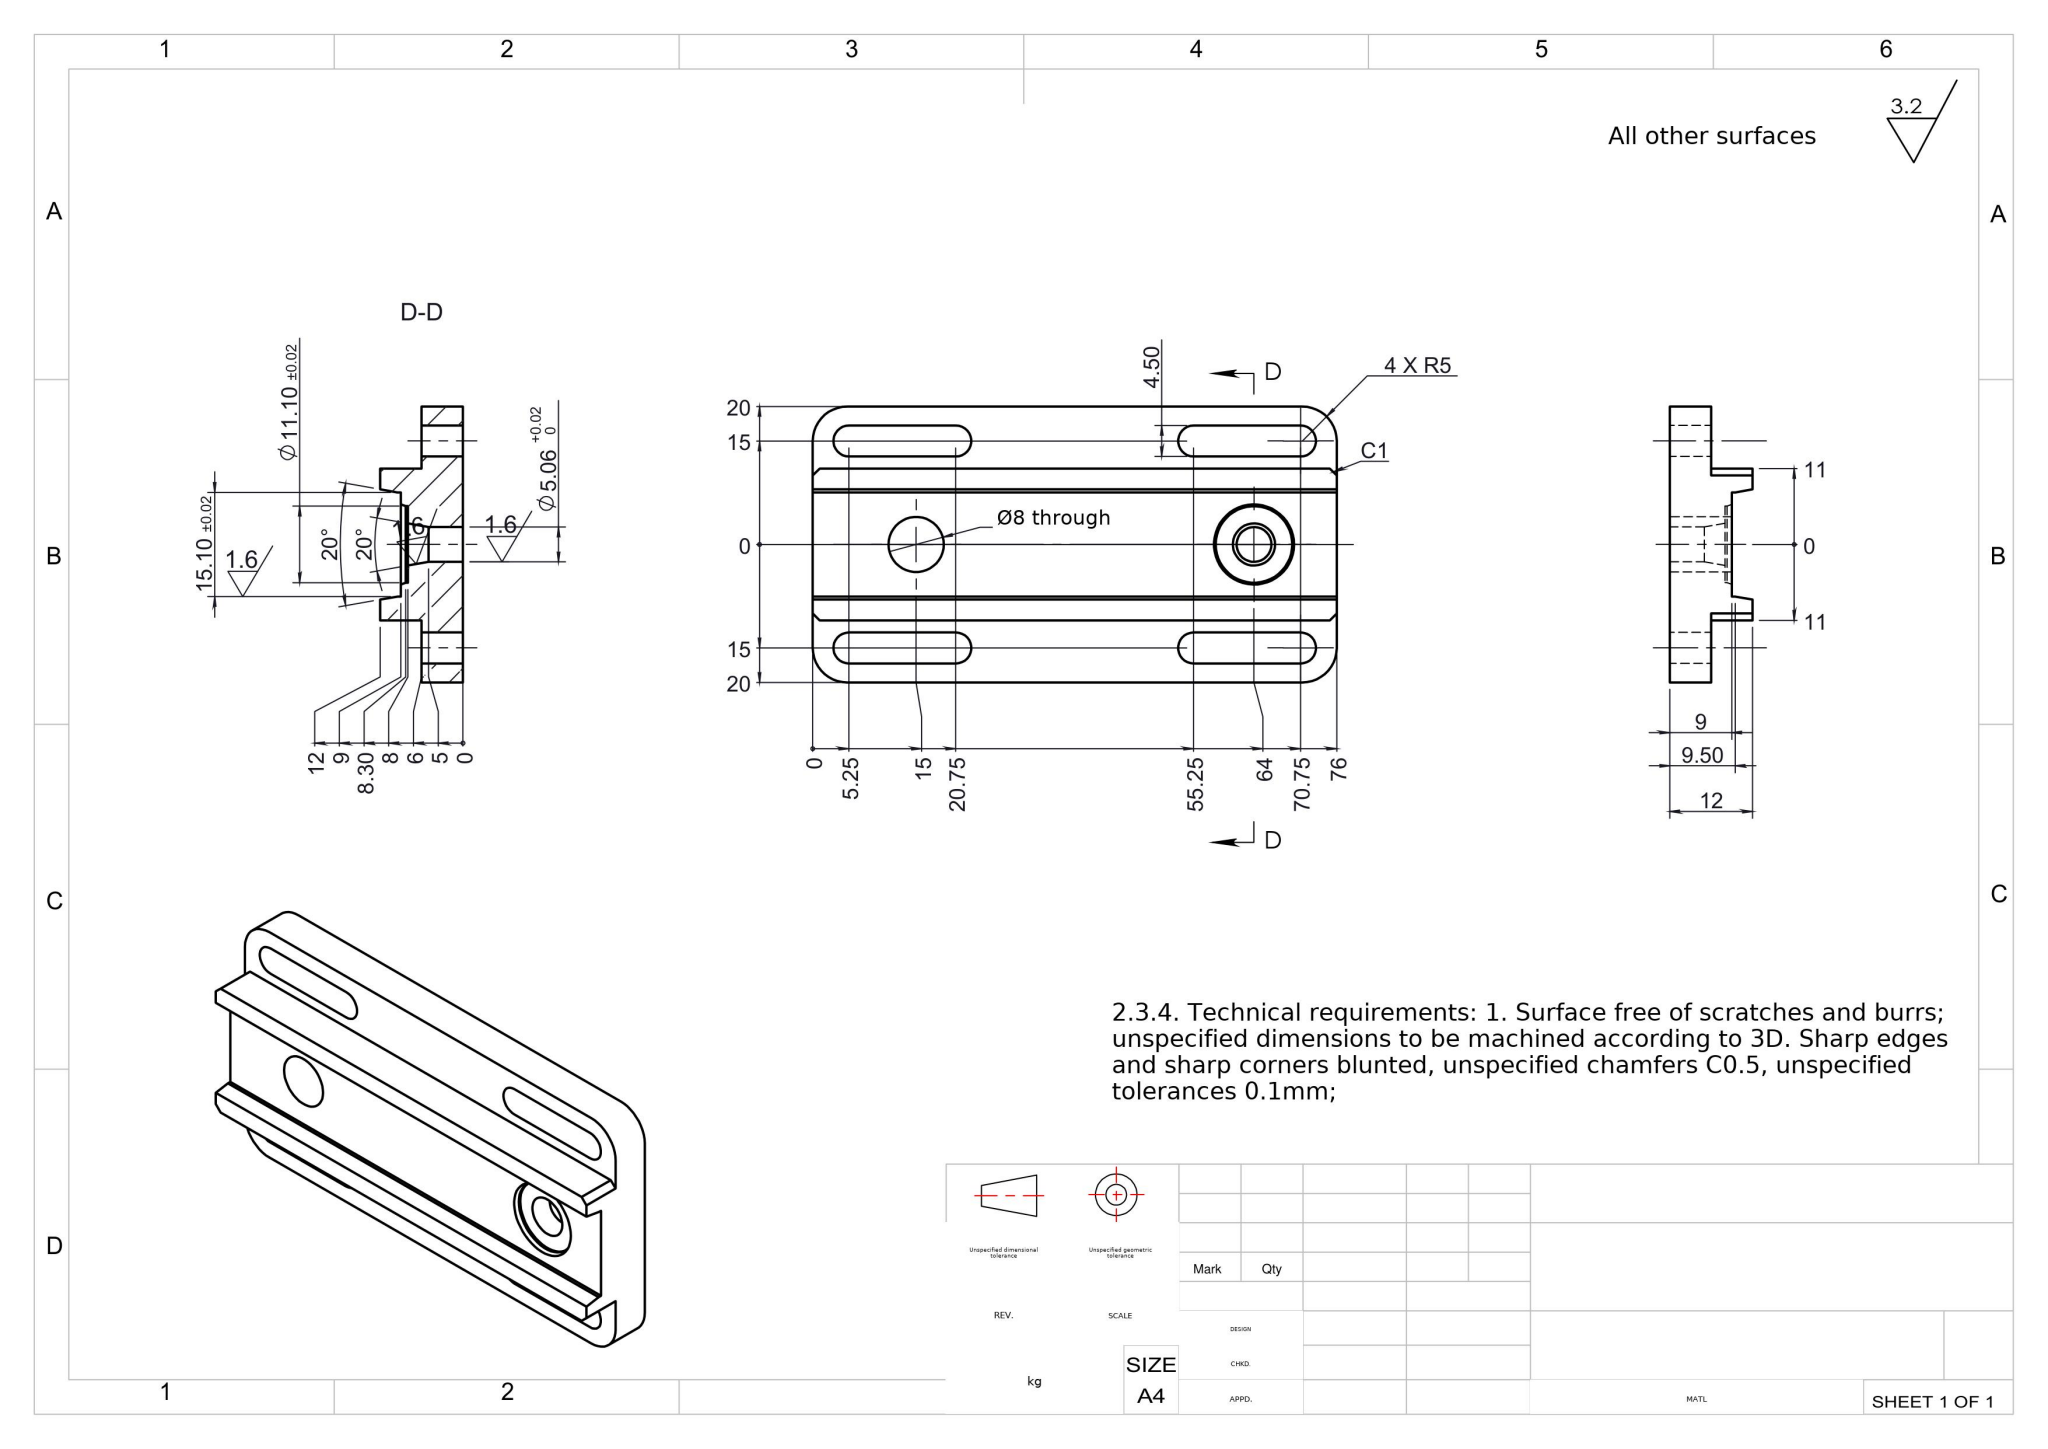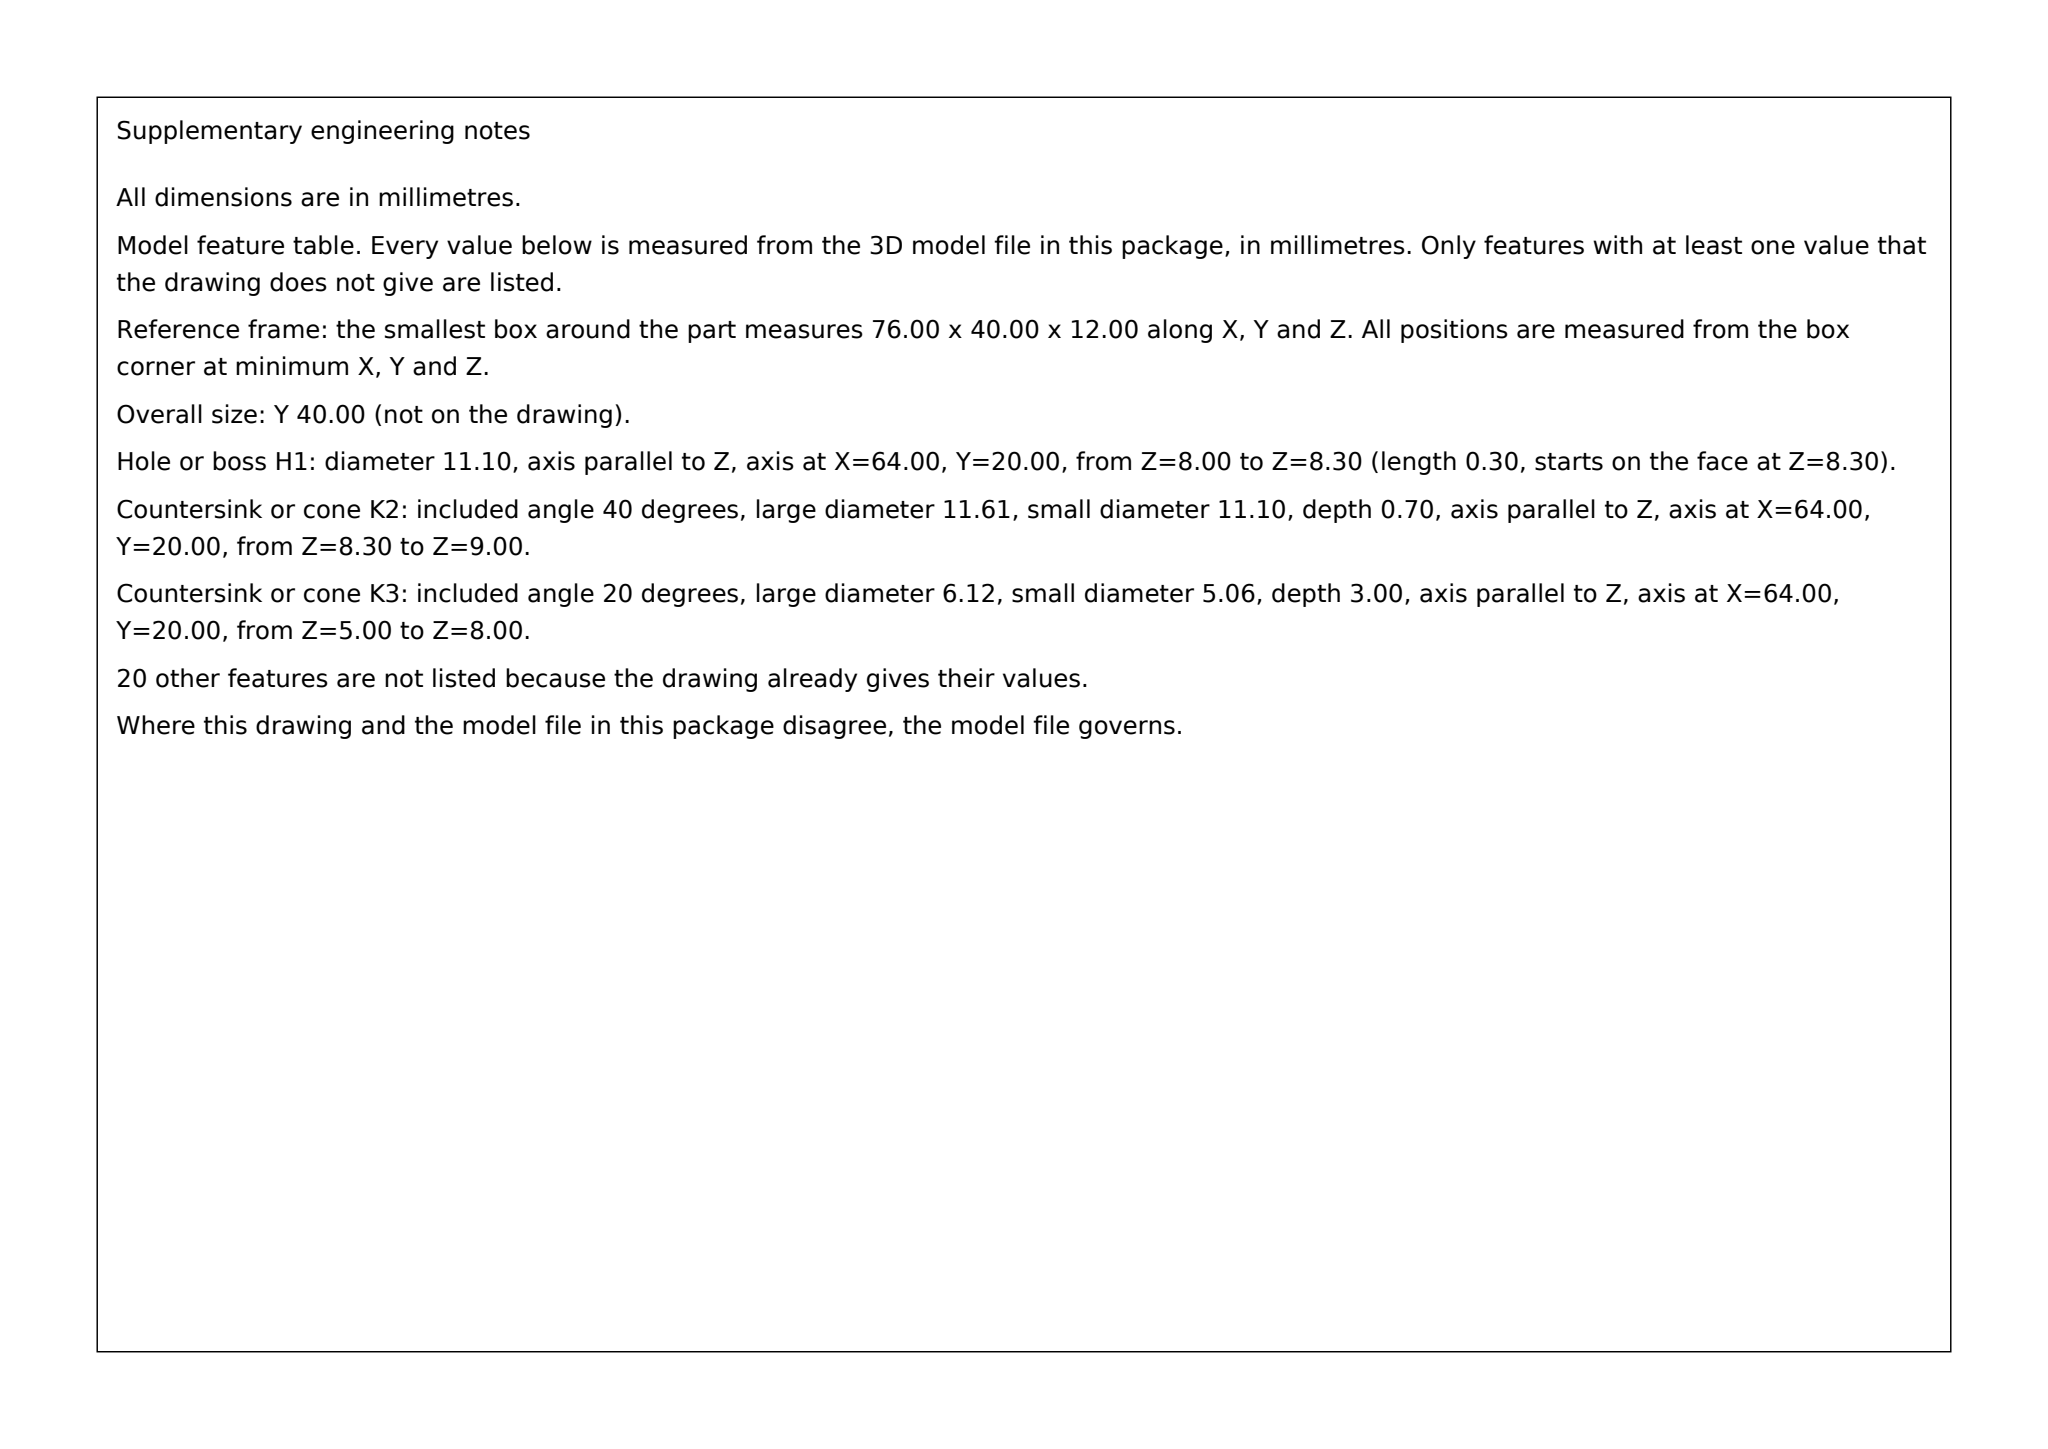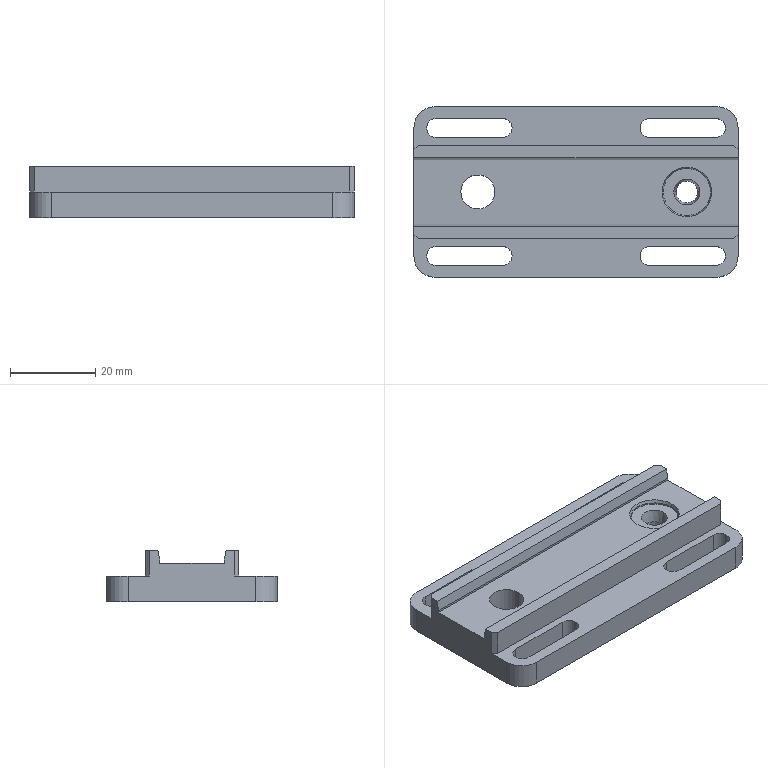Part | SolidWorks | mm | 1 solid | 55 faces | box 76 x 40 x 12 mm | volume 21822 mm3 | plane 29 | cylinder 22 | cone 4 | commonest cylinder face diameters 4.5 x12 10 x4 5.06 x2 8 x2 11.1 x2